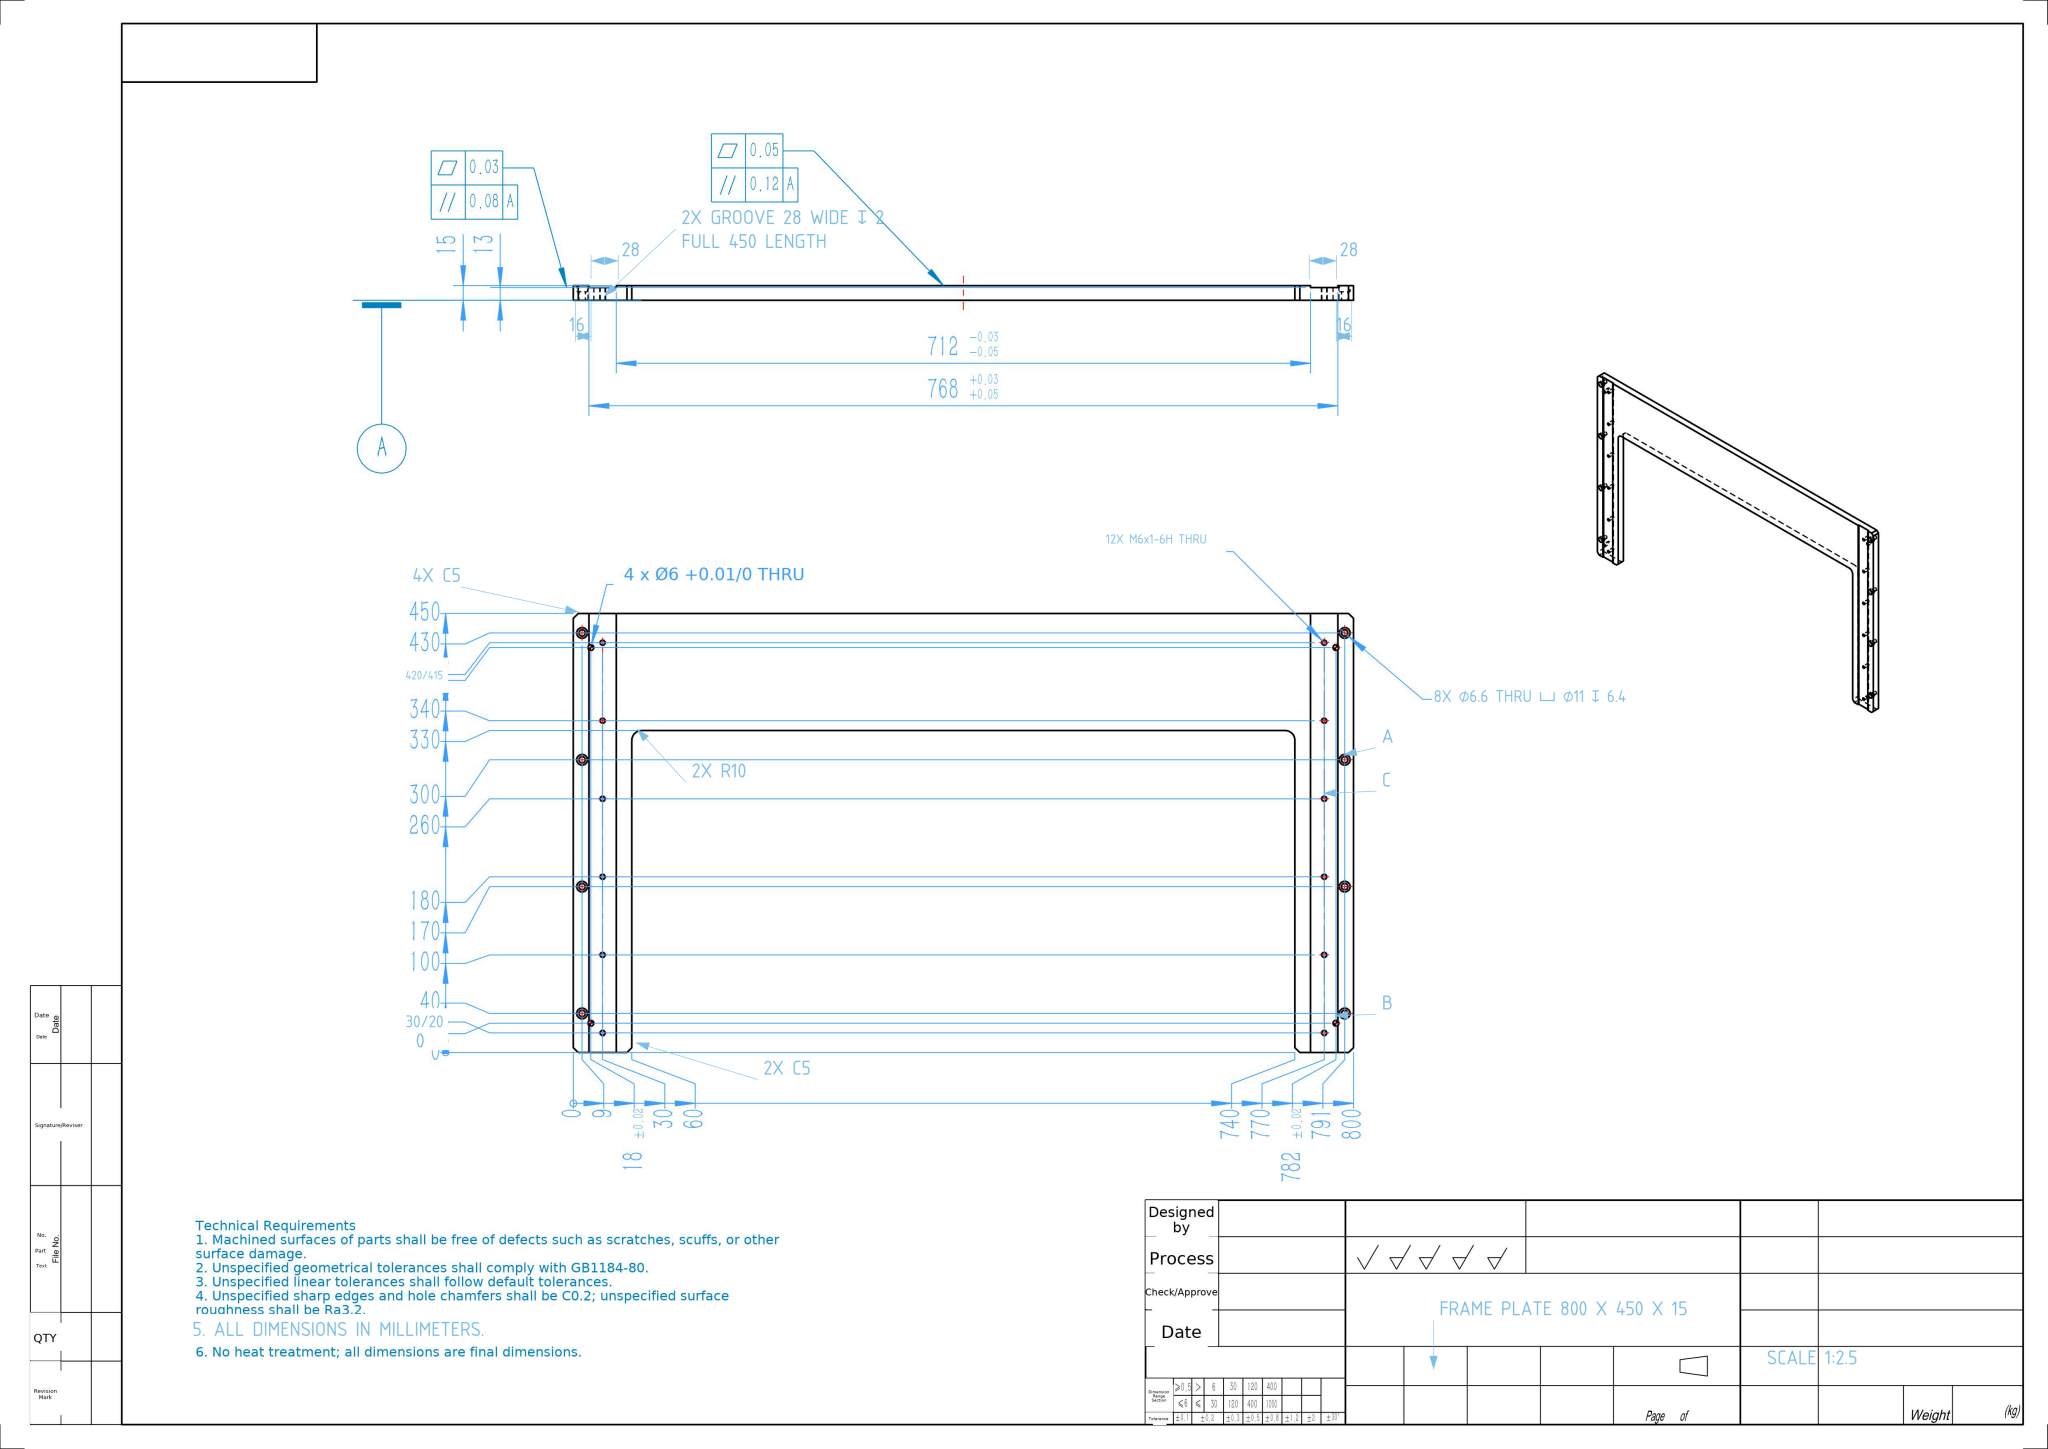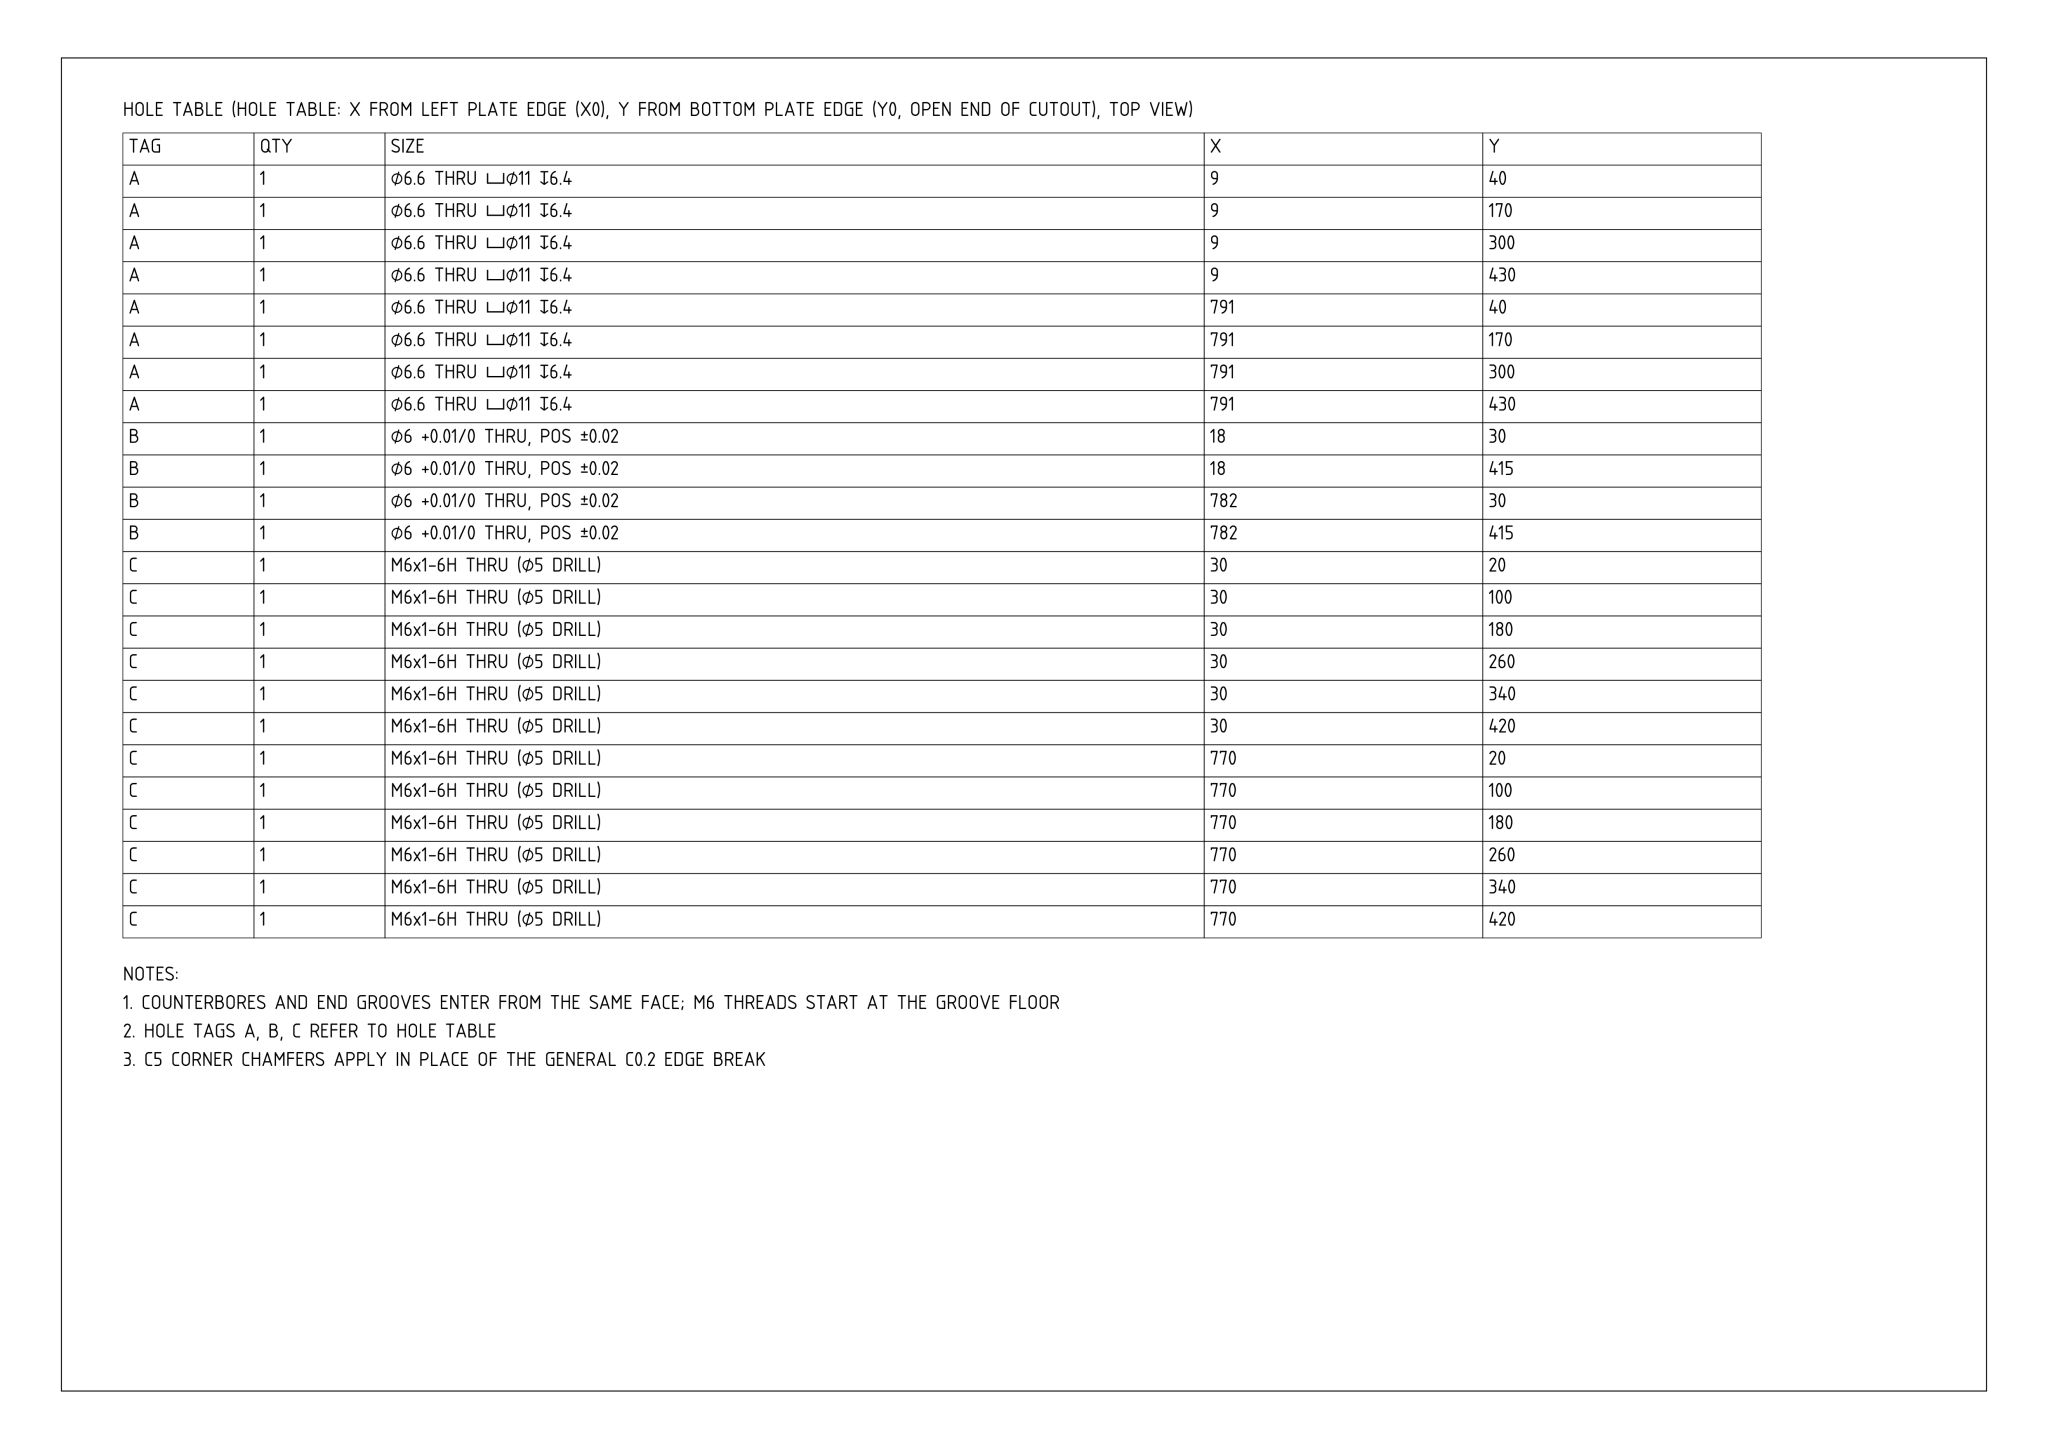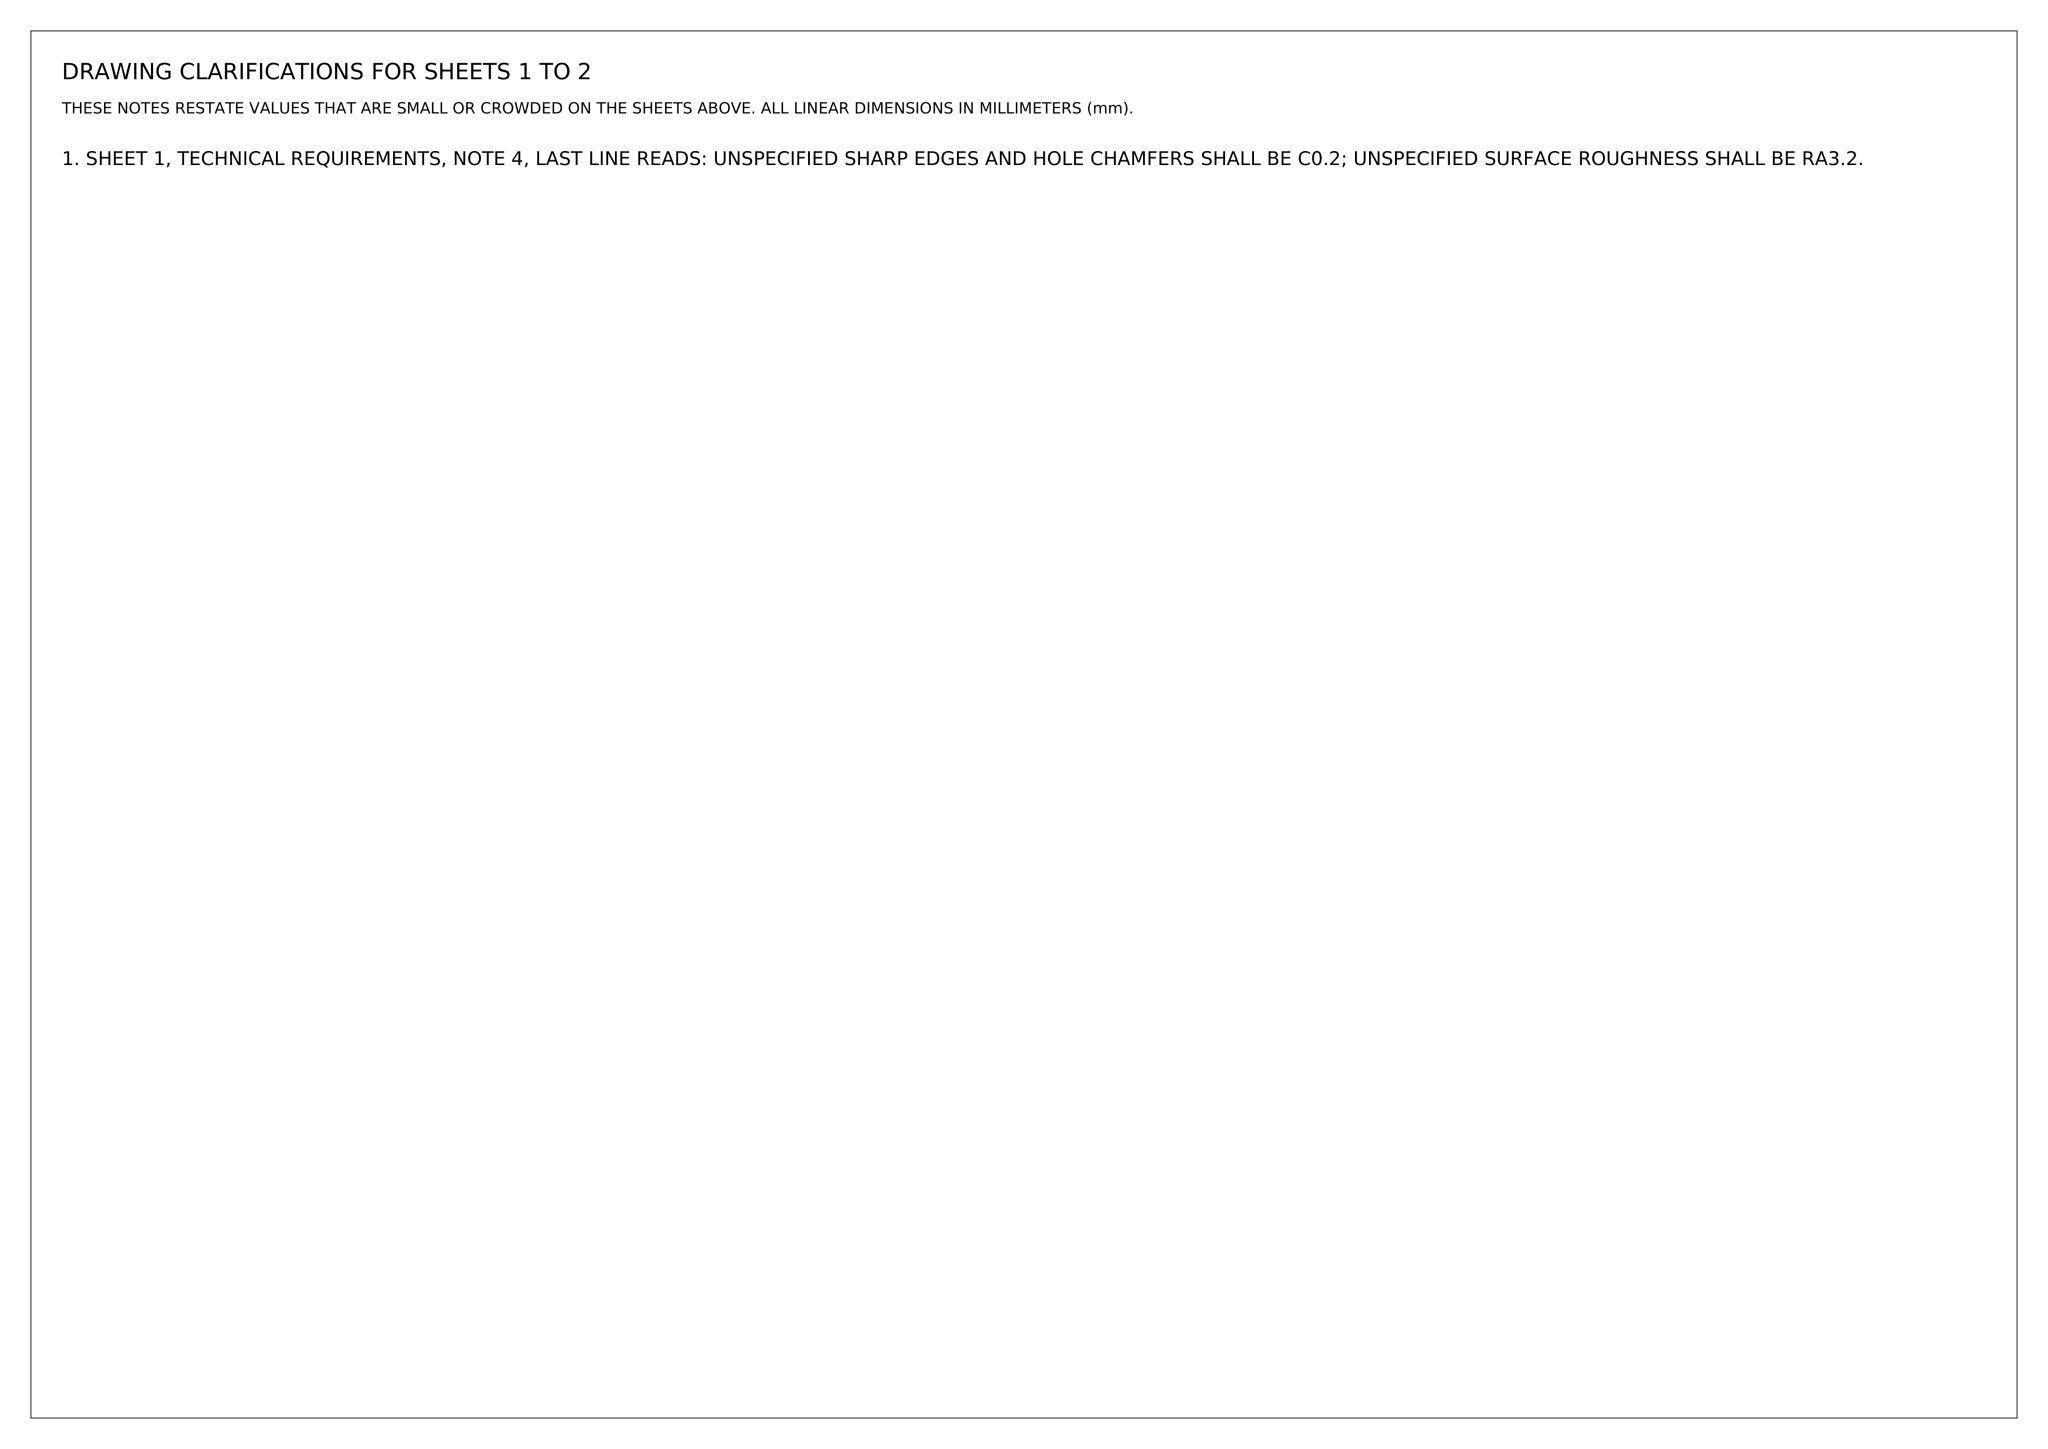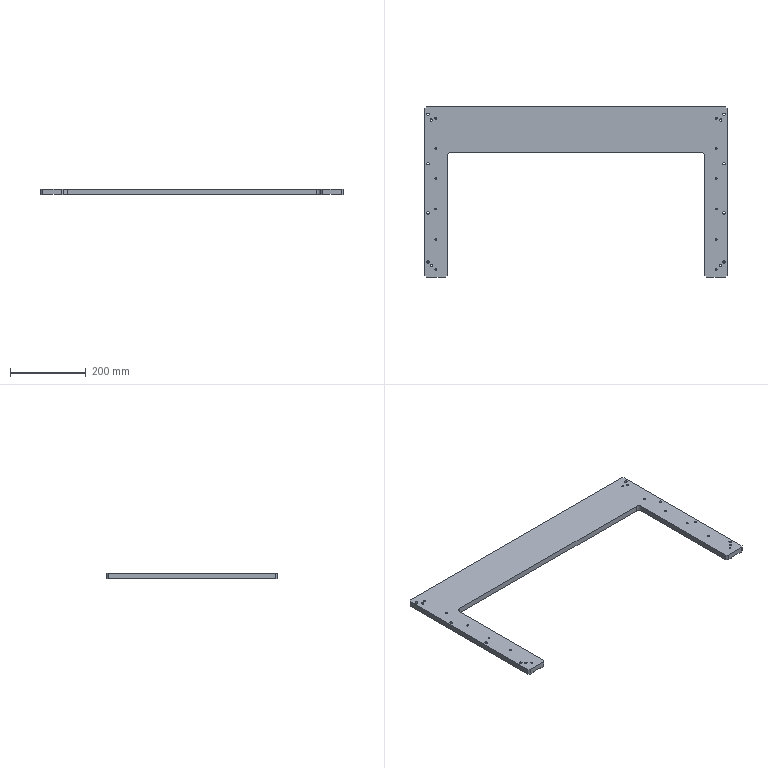Part | NX | mm | 1 solid | 102 faces | box 800 x 450 x 15 mm | volume 1971341 mm3 | cylinder 66 | plane 36 | commonest cylinder face diameters 5 x24 11 x16 6.6 x16 6 x8 20 x2